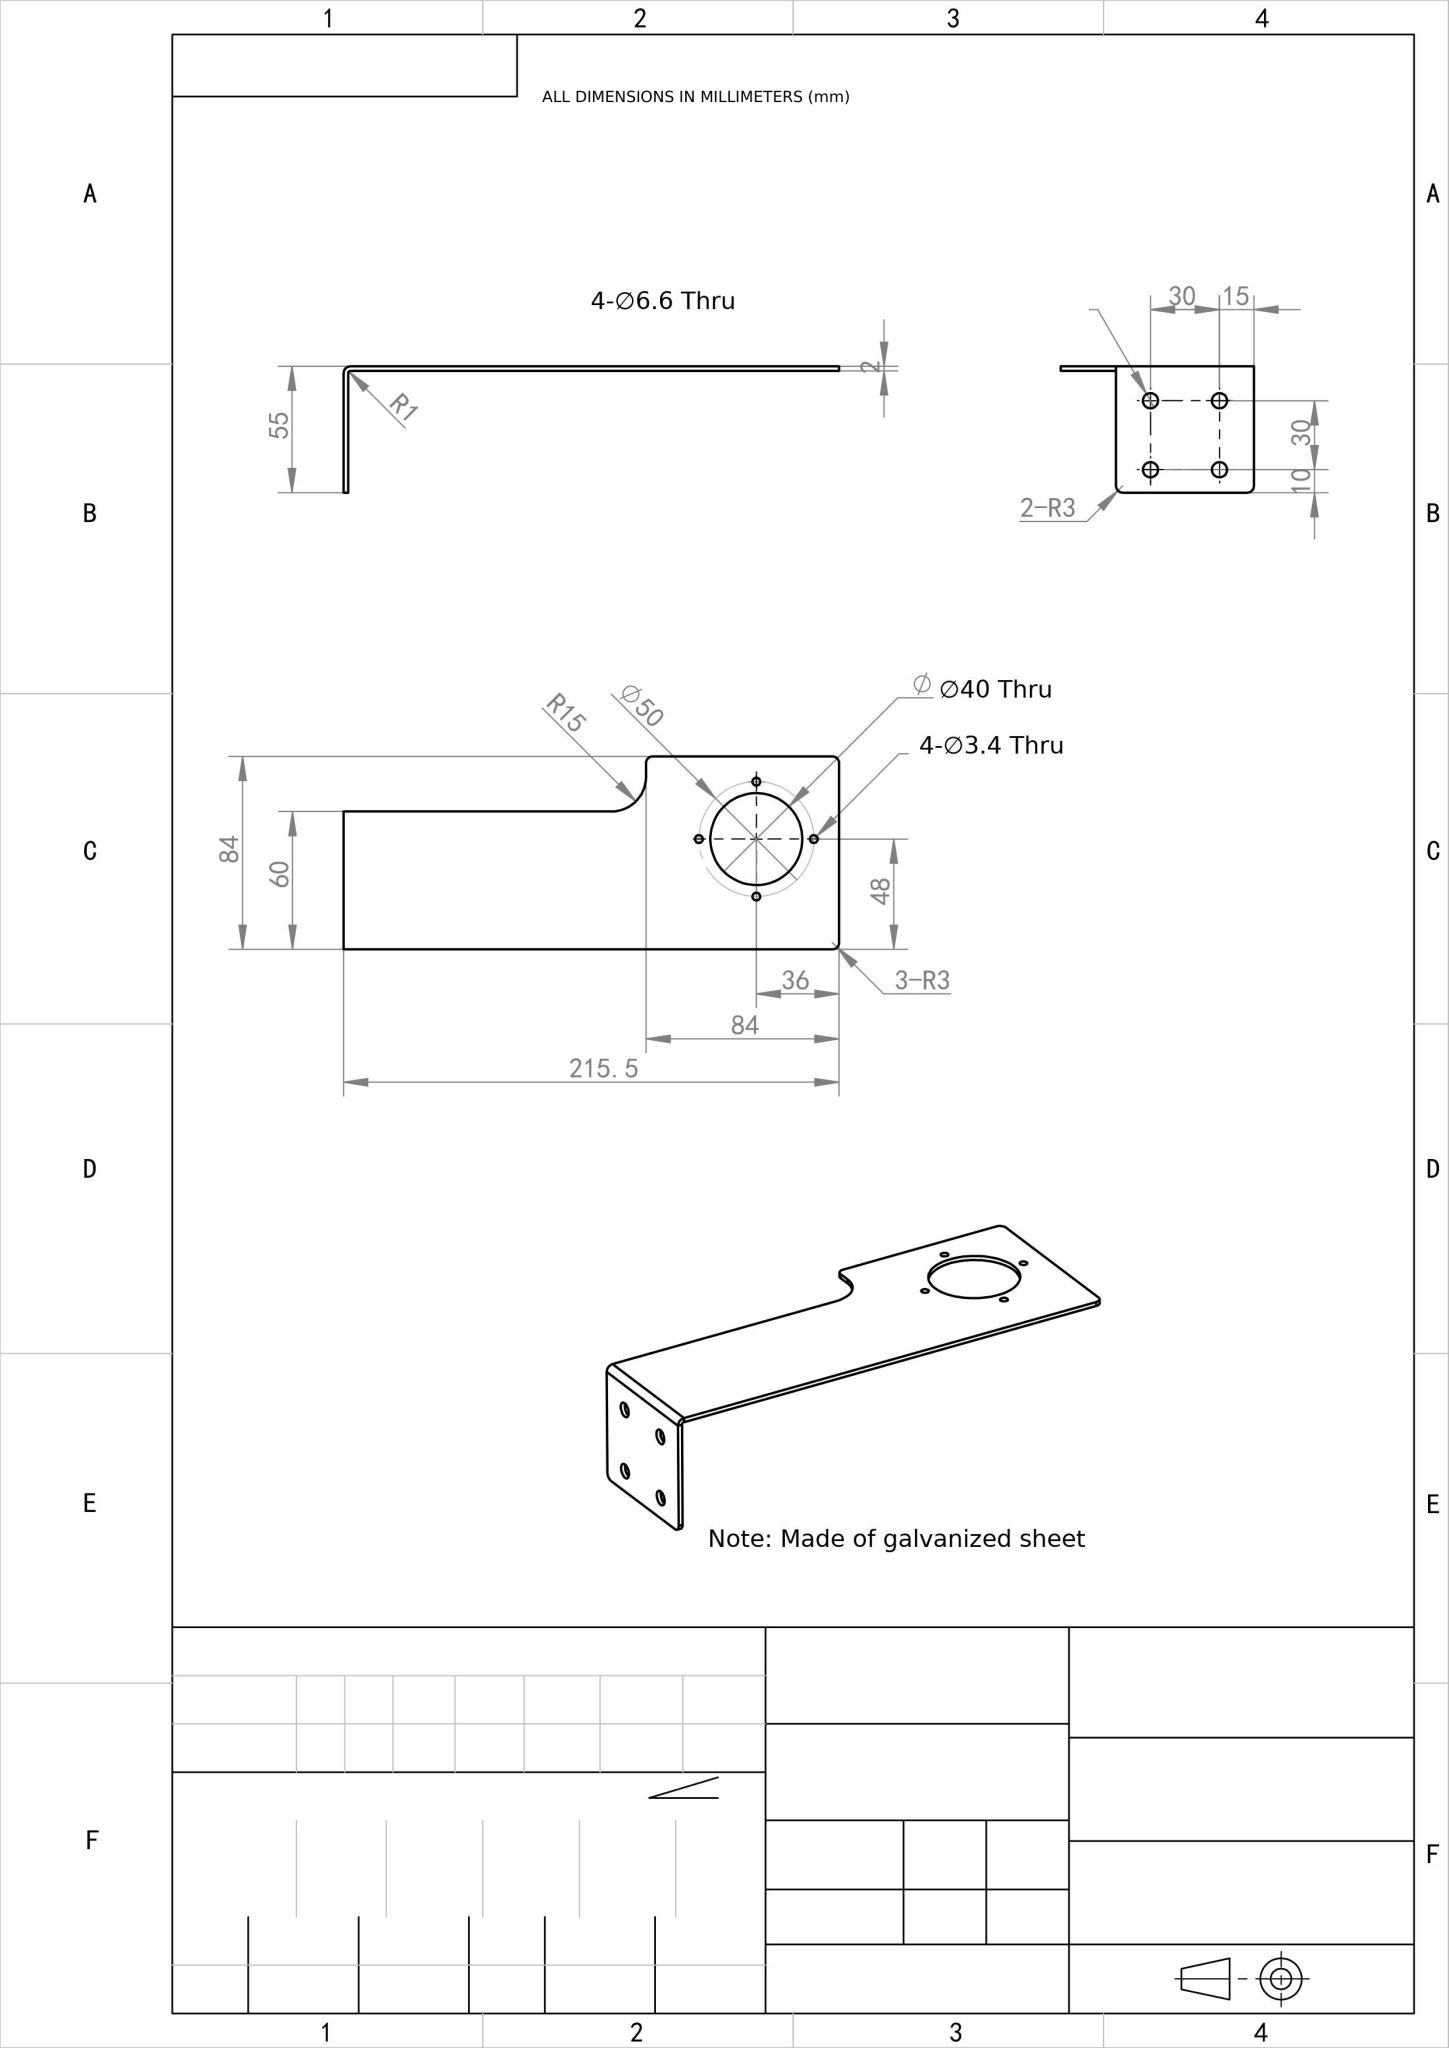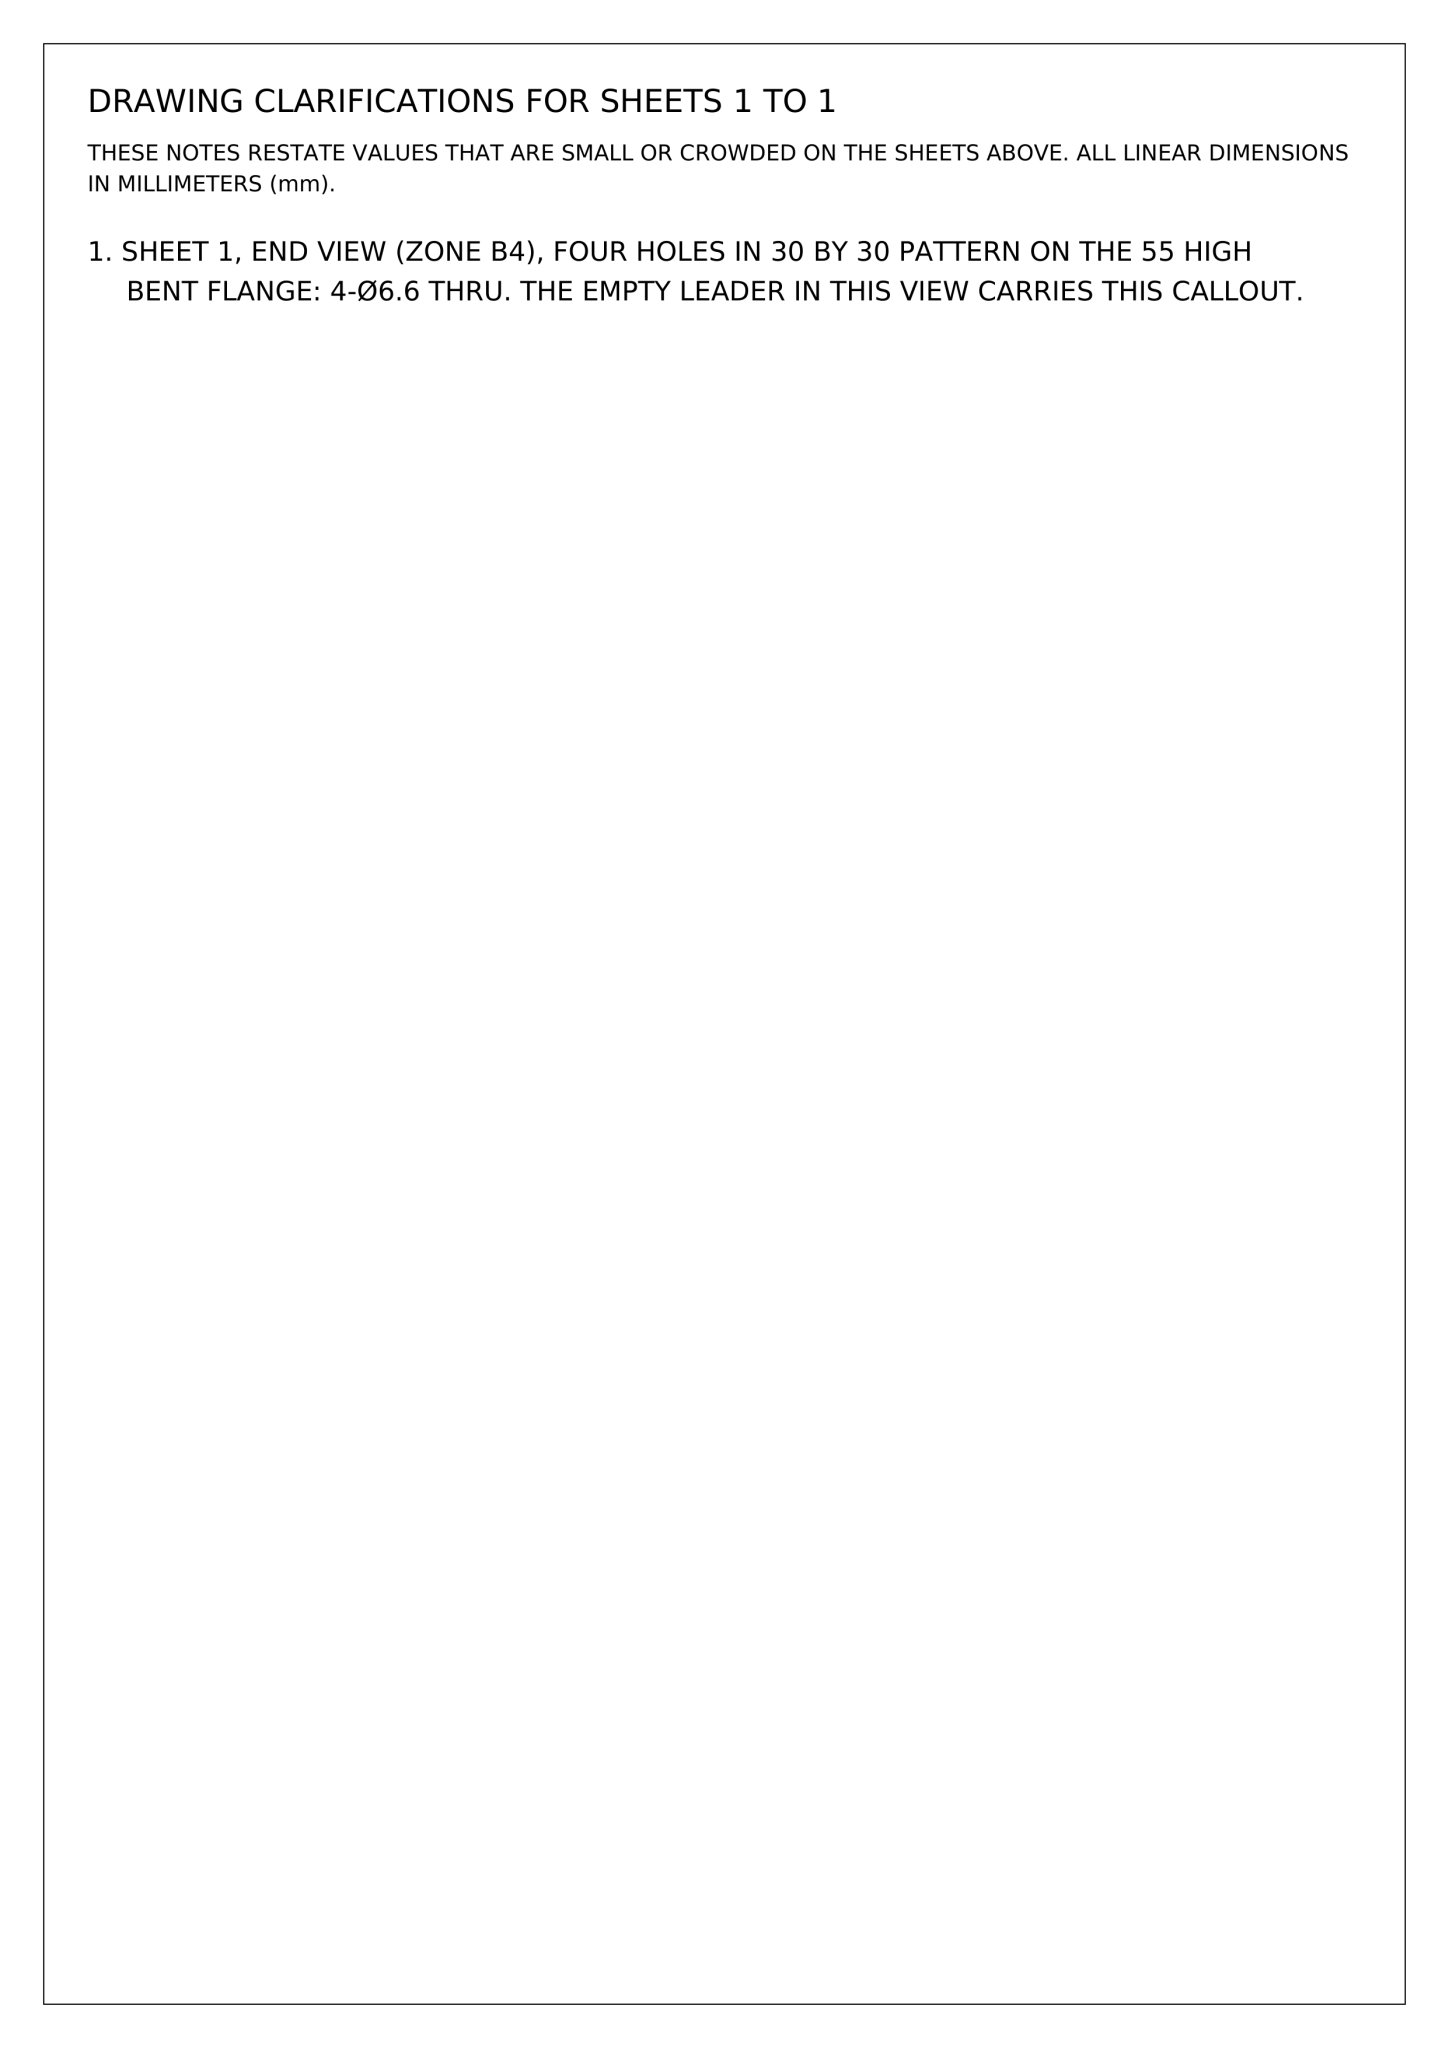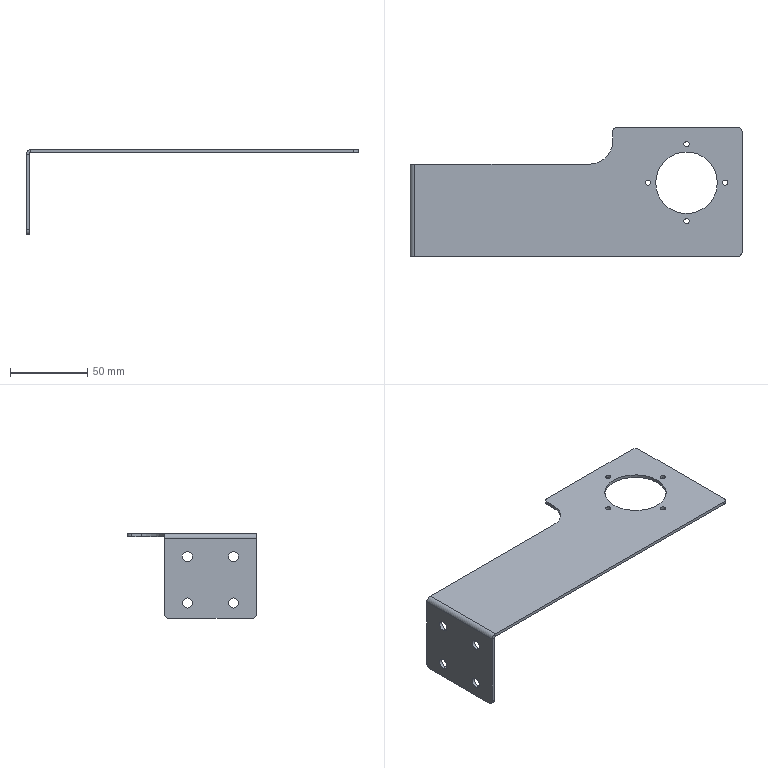Part | NX | mm | 1 solid | 40 faces | box 215.5 x 84 x 55 mm | volume 33367 mm3 | cylinder 26 | plane 14 | commonest cylinder face diameters 3.4 x8 6.6 x8 6 x6 40 x2 2 x1 30 x1